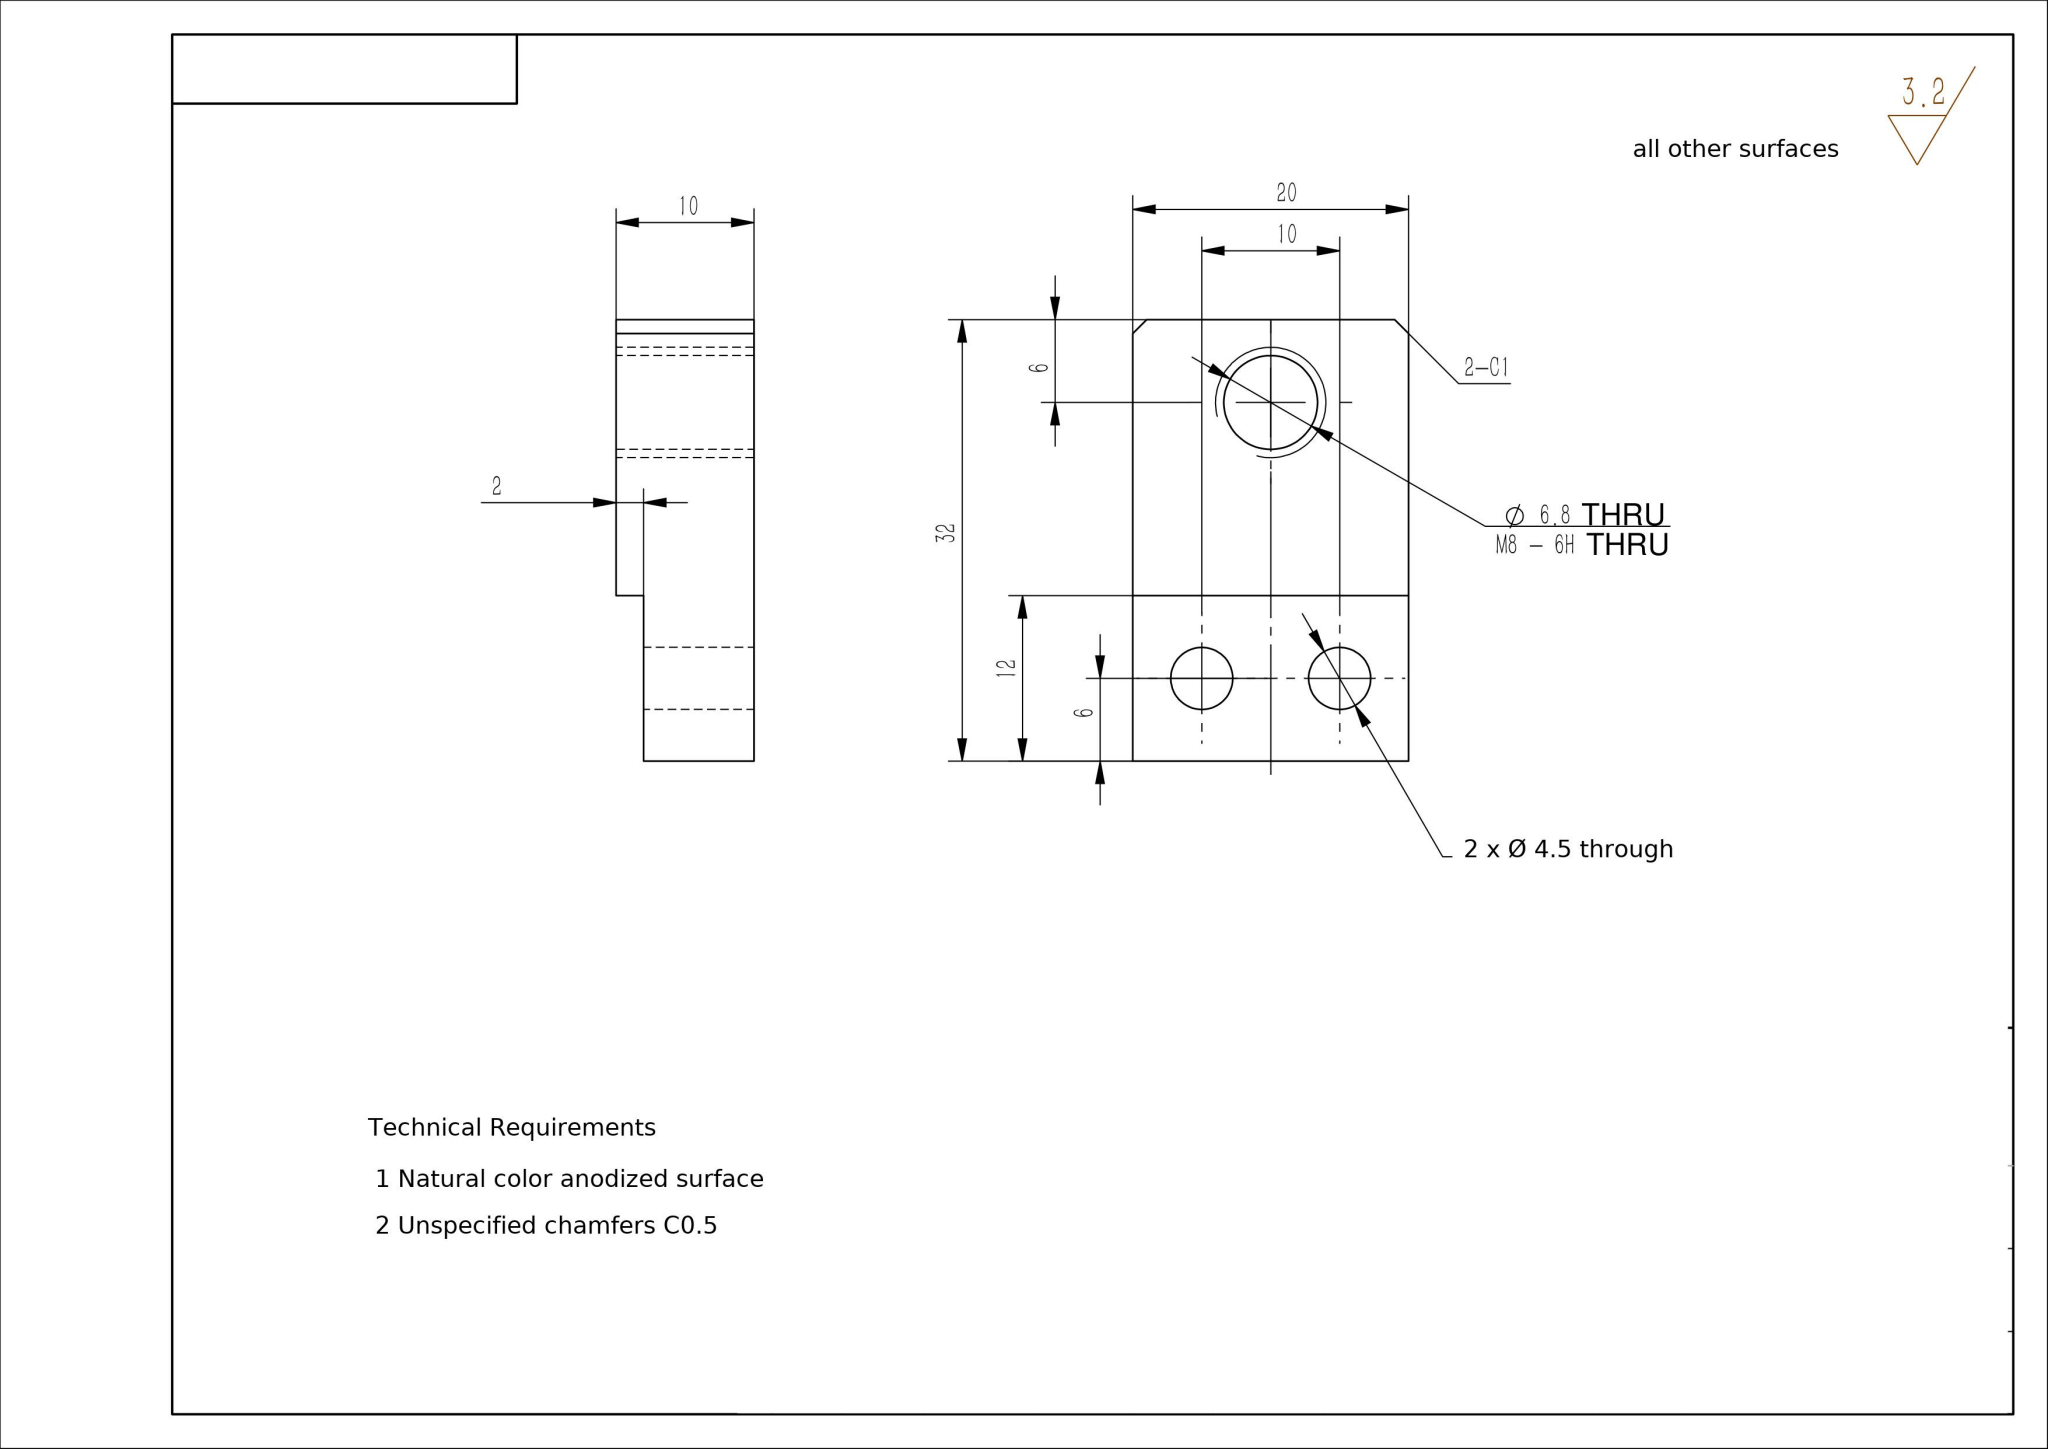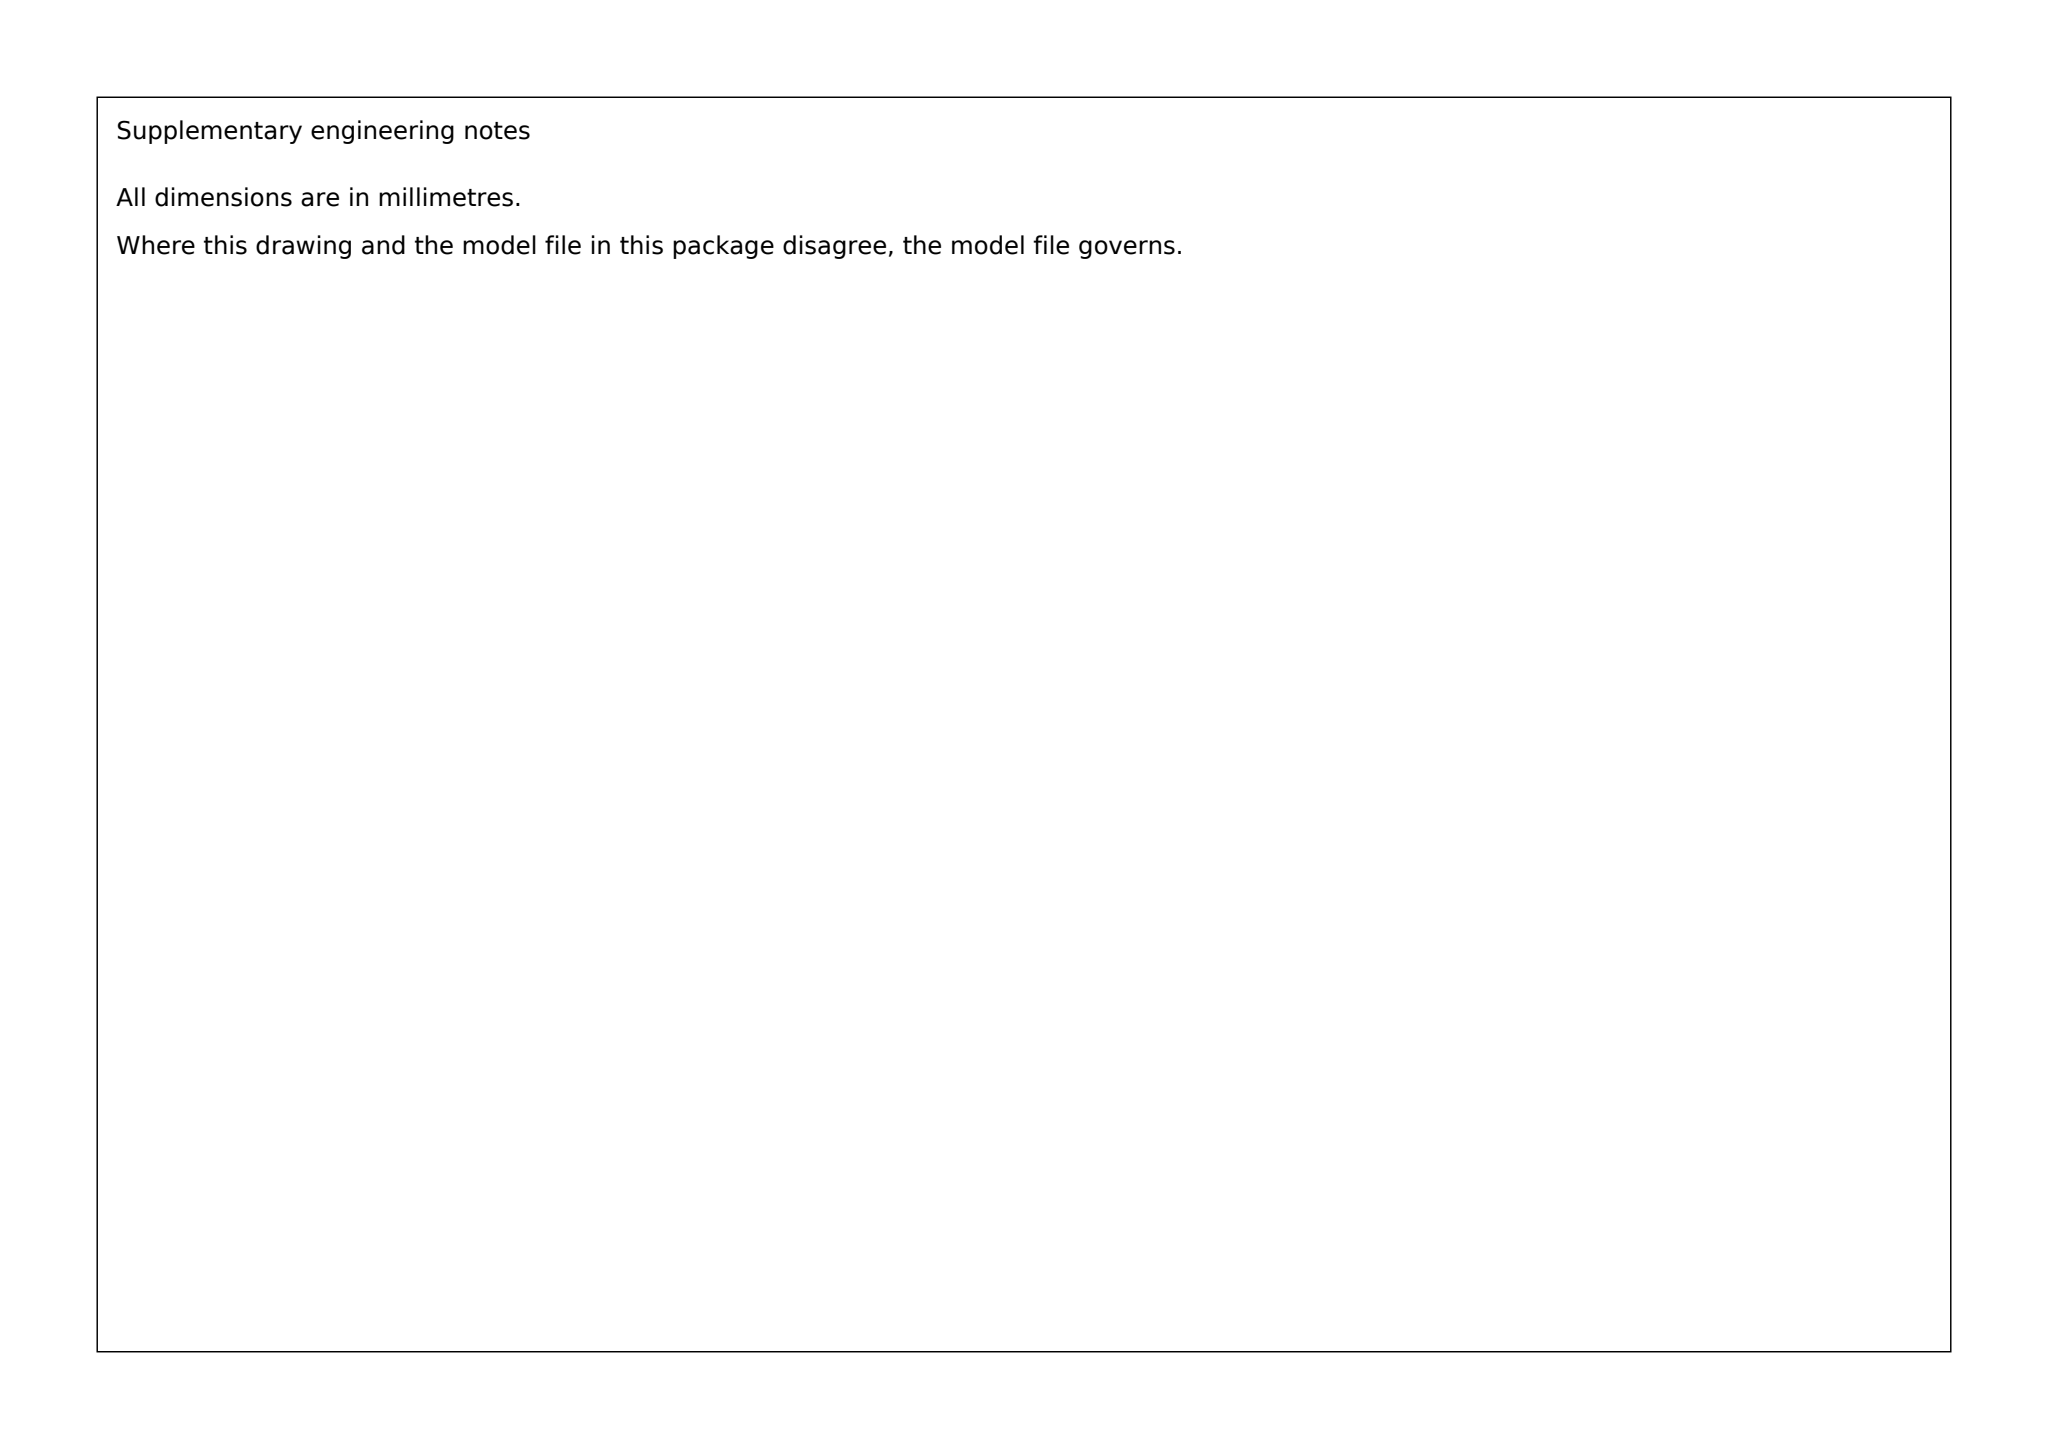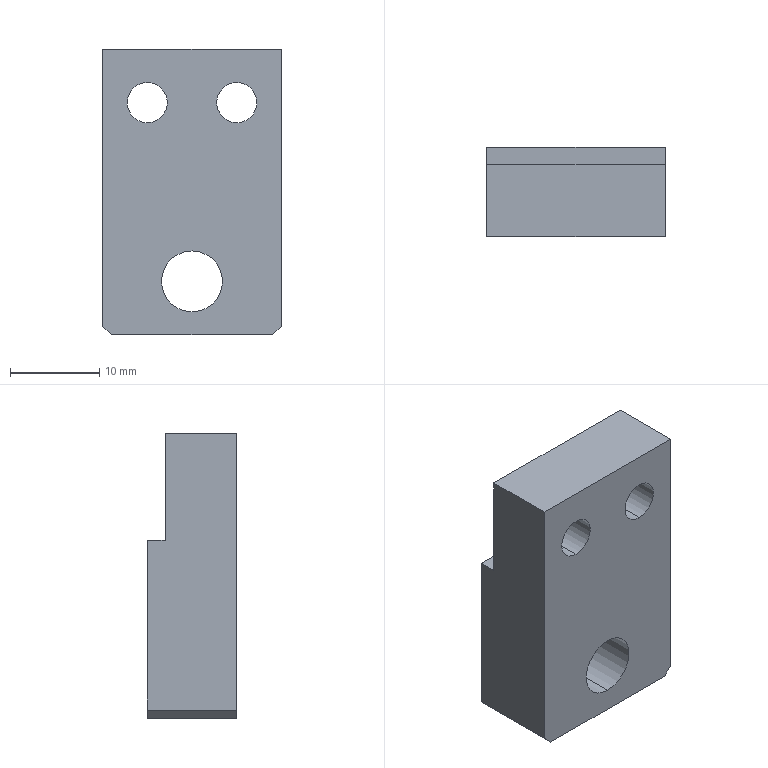Part | SolidWorks | mm | 1 solid | 16 faces | box 20 x 10 x 32 mm | volume 5292 mm3 | plane 10 | cylinder 6 | commonest cylinder face diameters 4.5 x4 6.8 x2
build123d program:
from build123d import *

# Parameters (mm, degrees)
SKETCH1_W                  = 20
SKETCH1_H                  = 32
BOSS_EXTRUDE1_DEPTH        = 10
F_4_5_4_5_DIAMETER_HOLE1_D = 4.5
SKETCH4_W                  = 20
SKETCH4_H                  = 12
CUT_EXTRUDE1_DEPTH         = 2
M8_TAPPED_HOLE1_D          = 6.8
CHAMFER1_SIZE              = 1


with BuildPart() as part:
    # Sketch1 → Boss-Extrude1 (new body)
    with BuildSketch(Plane(origin=(0, 0, 0), x_dir=(1, 0, 0), z_dir=(0, 1, 0))):
        Rectangle(SKETCH1_W, SKETCH1_H)
    extrude(amount=BOSS_EXTRUDE1_DEPTH)

    # 4.5 _4.5_ Diameter Hole1 (through all)
    with Locations(Plane(origin=(0, 10, 0), x_dir=(1, 0, 0), z_dir=(0, 1, 0))):
        with Locations((-5, -10), (5, -10)):
            Hole(F_4_5_4_5_DIAMETER_HOLE1_D / 2)

    # Sketch4 → Cut-Extrude1 (cut)
    with BuildSketch(Plane(origin=(0, 10, 0), x_dir=(1, 0, 0), z_dir=(0, 1, 0))):
        with Locations((0, -10)):
            Rectangle(SKETCH4_W, SKETCH4_H)
    extrude(amount=-CUT_EXTRUDE1_DEPTH, mode=Mode.SUBTRACT)

    # M8 Tapped Hole1 (through all)
    with Locations(Plane(origin=(0, 0, 0), x_dir=(-1, 0, 0), z_dir=(0, -1, 0))):
        with Locations((0, 10)):
            Hole(M8_TAPPED_HOLE1_D / 2)

    # Chamfer1
    chamfer1_edges = [part.edges().sort_by_distance(p)[0] for p in [
        (-10, 5, -16),
        (10, 5, -16),
    ]]
    chamfer(chamfer1_edges, length=CHAMFER1_SIZE)


solid = part.part
STEP:
#1=CARTESIAN_POINT('',(0.,10.,-6.6));
#2=VERTEX_POINT('',#1);
#3=CARTESIAN_POINT('',(0.,10.,-13.4));
#4=VERTEX_POINT('',#3);
#5=CARTESIAN_POINT('',(0.,10.,-10.));
#6=DIRECTION('',(0.,-1.,0.));
#7=DIRECTION('',(0.,0.,-1.));
#8=AXIS2_PLACEMENT_3D('',#5,#6,#7);
#9=CIRCLE('',#8,3.4);
#10=EDGE_CURVE('',#2,#4,#9,.T.);
#11=ORIENTED_EDGE('',*,*,#10,.F.);
#12=CARTESIAN_POINT('',(0.,0.,-6.6));
#13=VERTEX_POINT('',#12);
#14=CARTESIAN_POINT('',(0.,0.,-6.6));
#15=DIRECTION('',(0.,-1.,0.));
#16=VECTOR('',#15,1000.);
#17=LINE('',#14,#16);
#18=EDGE_CURVE('',#2,#13,#17,.T.);
#19=ORIENTED_EDGE('',*,*,#18,.T.);
#20=CARTESIAN_POINT('',(0.,0.,-13.4));
#21=VERTEX_POINT('',#20);
#22=CARTESIAN_POINT('',(0.,0.,-10.));
#23=DIRECTION('',(0.,-1.,0.));
#24=DIRECTION('',(0.,0.,-1.));
#25=AXIS2_PLACEMENT_3D('',#22,#23,#24);
#26=CIRCLE('',#25,3.4);
#27=EDGE_CURVE('',#13,#21,#26,.T.);
#28=ORIENTED_EDGE('',*,*,#27,.T.);
#29=CARTESIAN_POINT('',(0.,0.,-13.4));
#30=DIRECTION('',(0.,-1.,0.));
#31=VECTOR('',#30,1000.);
#32=LINE('',#29,#31);
#33=EDGE_CURVE('',#4,#21,#32,.T.);
#34=ORIENTED_EDGE('',*,*,#33,.F.);
#35=EDGE_LOOP('',(#11,#19,#28,#34));
#36=FACE_OUTER_BOUND('',#35,.T.);
#37=CARTESIAN_POINT('',(0.,0.,-10.));
#38=DIRECTION('',(0.,-1.,0.));
#39=DIRECTION('',(0.,0.,-1.));
#40=AXIS2_PLACEMENT_3D('',#37,#38,#39);
#41=CYLINDRICAL_SURFACE('',#40,3.4);
#42=ADVANCED_FACE('',(#36),#41,.F.);
#43=CARTESIAN_POINT('',(-5.,0.,7.75));
#44=VERTEX_POINT('',#43);
#45=CARTESIAN_POINT('',(-5.,0.,12.25));
#46=VERTEX_POINT('',#45);
#47=CARTESIAN_POINT('',(-5.,0.,10.));
#48=DIRECTION('',(0.,1.,0.));
#49=DIRECTION('',(0.,0.,1.));
#50=AXIS2_PLACEMENT_3D('',#47,#48,#49);
#51=CIRCLE('',#50,2.25);
#52=EDGE_CURVE('',#44,#46,#51,.T.);
#53=ORIENTED_EDGE('',*,*,#52,.F.);
#54=CARTESIAN_POINT('',(-5.,8.,7.75));
#55=VERTEX_POINT('',#54);
#56=CARTESIAN_POINT('',(-5.,10.,7.75));
#57=DIRECTION('',(0.,1.,0.));
#58=VECTOR('',#57,1000.);
#59=LINE('',#56,#58);
#60=EDGE_CURVE('',#44,#55,#59,.T.);
#61=ORIENTED_EDGE('',*,*,#60,.T.);
#62=CARTESIAN_POINT('',(-5.,8.,12.25));
#63=VERTEX_POINT('',#62);
#64=CARTESIAN_POINT('',(-5.,8.,10.));
#65=DIRECTION('',(0.,-1.,0.));
#66=DIRECTION('',(0.,0.,1.));
#67=AXIS2_PLACEMENT_3D('',#64,#65,#66);
#68=CIRCLE('',#67,2.25);
#69=EDGE_CURVE('',#63,#55,#68,.T.);
#70=ORIENTED_EDGE('',*,*,#69,.F.);
#71=CARTESIAN_POINT('',(-5.,10.,12.25));
#72=DIRECTION('',(0.,1.,0.));
#73=VECTOR('',#72,1000.);
#74=LINE('',#71,#73);
#75=EDGE_CURVE('',#46,#63,#74,.T.);
#76=ORIENTED_EDGE('',*,*,#75,.F.);
#77=EDGE_LOOP('',(#53,#61,#70,#76));
#78=FACE_OUTER_BOUND('',#77,.T.);
#79=CARTESIAN_POINT('',(-5.,10.,10.));
#80=DIRECTION('',(0.,1.,0.));
#81=DIRECTION('',(0.,0.,1.));
#82=AXIS2_PLACEMENT_3D('',#79,#80,#81);
#83=CYLINDRICAL_SURFACE('',#82,2.25);
#84=ADVANCED_FACE('',(#78),#83,.F.);
#85=CARTESIAN_POINT('',(5.,0.,7.75));
#86=VERTEX_POINT('',#85);
#87=CARTESIAN_POINT('',(5.,0.,12.25));
#88=VERTEX_POINT('',#87);
#89=CARTESIAN_POINT('',(5.,0.,10.));
#90=DIRECTION('',(0.,1.,0.));
#91=DIRECTION('',(0.,0.,1.));
#92=AXIS2_PLACEMENT_3D('',#89,#90,#91);
#93=CIRCLE('',#92,2.25);
#94=EDGE_CURVE('',#86,#88,#93,.T.);
#95=ORIENTED_EDGE('',*,*,#94,.F.);
#96=CARTESIAN_POINT('',(5.,8.,7.75));
#97=VERTEX_POINT('',#96);
#98=CARTESIAN_POINT('',(5.,10.,7.75));
#99=DIRECTION('',(0.,1.,0.));
#100=VECTOR('',#99,1000.);
#101=LINE('',#98,#100);
#102=EDGE_CURVE('',#86,#97,#101,.T.);
#103=ORIENTED_EDGE('',*,*,#102,.T.);
#104=CARTESIAN_POINT('',(5.,8.,12.25));
#105=VERTEX_POINT('',#104);
#106=CARTESIAN_POINT('',(5.,8.,10.));
#107=DIRECTION('',(0.,-1.,0.));
#108=DIRECTION('',(0.,0.,1.));
#109=AXIS2_PLACEMENT_3D('',#106,#107,#108);
#110=CIRCLE('',#109,2.25);
#111=EDGE_CURVE('',#105,#97,#110,.T.);
#112=ORIENTED_EDGE('',*,*,#111,.F.);
#113=CARTESIAN_POINT('',(5.,10.,12.25));
#114=DIRECTION('',(0.,1.,0.));
#115=VECTOR('',#114,1000.);
#116=LINE('',#113,#115);
#117=EDGE_CURVE('',#88,#105,#116,.T.);
#118=ORIENTED_EDGE('',*,*,#117,.F.);
#119=EDGE_LOOP('',(#95,#103,#112,#118));
#120=FACE_OUTER_BOUND('',#119,.T.);
#121=CARTESIAN_POINT('',(5.,10.,10.));
#122=DIRECTION('',(0.,1.,0.));
#123=DIRECTION('',(0.,0.,1.));
#124=AXIS2_PLACEMENT_3D('',#121,#122,#123);
#125=CYLINDRICAL_SURFACE('',#124,2.25);
#126=ADVANCED_FACE('',(#120),#125,.F.);
#127=CARTESIAN_POINT('',(-10.,8.,16.));
#128=VERTEX_POINT('',#127);
#129=CARTESIAN_POINT('',(10.,8.,16.));
#130=VERTEX_POINT('',#129);
#131=CARTESIAN_POINT('',(-10.,8.,16.));
#132=DIRECTION('',(1.,0.,0.));
#133=VECTOR('',#132,1000.);
#134=LINE('',#131,#133);
#135=EDGE_CURVE('',#128,#130,#134,.T.);
#136=ORIENTED_EDGE('',*,*,#135,.F.);
#137=CARTESIAN_POINT('',(-10.,0.,16.));
#138=VERTEX_POINT('',#137);
#139=CARTESIAN_POINT('',(-10.,10.,16.));
#140=DIRECTION('',(0.,-1.,0.));
#141=VECTOR('',#140,1000.);
#142=LINE('',#139,#141);
#143=EDGE_CURVE('',#128,#138,#142,.T.);
#144=ORIENTED_EDGE('',*,*,#143,.T.);
#145=CARTESIAN_POINT('',(10.,0.,16.));
#146=VERTEX_POINT('',#145);
#147=CARTESIAN_POINT('',(-10.,0.,16.));
#148=DIRECTION('',(1.,0.,0.));
#149=VECTOR('',#148,1000.);
#150=LINE('',#147,#149);
#151=EDGE_CURVE('',#138,#146,#150,.T.);
#152=ORIENTED_EDGE('',*,*,#151,.T.);
#153=CARTESIAN_POINT('',(10.,10.,16.));
#154=DIRECTION('',(0.,-1.,0.));
#155=VECTOR('',#154,1000.);
#156=LINE('',#153,#155);
#157=EDGE_CURVE('',#130,#146,#156,.T.);
#158=ORIENTED_EDGE('',*,*,#157,.F.);
#159=EDGE_LOOP('',(#136,#144,#152,#158));
#160=FACE_OUTER_BOUND('',#159,.T.);
#161=CARTESIAN_POINT('',(-10.,10.,16.));
#162=DIRECTION('',(0.,0.,-1.));
#163=DIRECTION('',(-1.,0.,0.));
#164=AXIS2_PLACEMENT_3D('',#161,#162,#163);
#165=PLANE('',#164);
#166=ADVANCED_FACE('',(#160),#165,.F.);
#167=ORIENTED_EDGE('',*,*,#102,.F.);
#168=CARTESIAN_POINT('',(5.,0.,10.));
#169=DIRECTION('',(0.,1.,0.));
#170=DIRECTION('',(0.,0.,1.));
#171=AXIS2_PLACEMENT_3D('',#168,#169,#170);
#172=CIRCLE('',#171,2.25);
#173=EDGE_CURVE('',#88,#86,#172,.T.);
#174=ORIENTED_EDGE('',*,*,#173,.F.);
#175=ORIENTED_EDGE('',*,*,#117,.T.);
#176=CARTESIAN_POINT('',(5.,8.,10.));
#177=DIRECTION('',(0.,-1.,0.));
#178=DIRECTION('',(0.,0.,1.));
#179=AXIS2_PLACEMENT_3D('',#176,#177,#178);
#180=CIRCLE('',#179,2.25);
#181=EDGE_CURVE('',#97,#105,#180,.T.);
#182=ORIENTED_EDGE('',*,*,#181,.F.);
#183=EDGE_LOOP('',(#167,#174,#175,#182));
#184=FACE_OUTER_BOUND('',#183,.T.);
#185=CARTESIAN_POINT('',(5.,10.,10.));
#186=DIRECTION('',(0.,1.,0.));
#187=DIRECTION('',(0.,0.,1.));
#188=AXIS2_PLACEMENT_3D('',#185,#186,#187);
#189=CYLINDRICAL_SURFACE('',#188,2.25);
#190=ADVANCED_FACE('',(#184),#189,.F.);
#191=ORIENTED_EDGE('',*,*,#60,.F.);
#192=CARTESIAN_POINT('',(-5.,0.,10.));
#193=DIRECTION('',(0.,1.,0.));
#194=DIRECTION('',(0.,0.,1.));
#195=AXIS2_PLACEMENT_3D('',#192,#193,#194);
#196=CIRCLE('',#195,2.25);
#197=EDGE_CURVE('',#46,#44,#196,.T.);
#198=ORIENTED_EDGE('',*,*,#197,.F.);
#199=ORIENTED_EDGE('',*,*,#75,.T.);
#200=CARTESIAN_POINT('',(-5.,8.,10.));
#201=DIRECTION('',(0.,-1.,0.));
#202=DIRECTION('',(0.,0.,1.));
#203=AXIS2_PLACEMENT_3D('',#200,#201,#202);
#204=CIRCLE('',#203,2.25);
#205=EDGE_CURVE('',#55,#63,#204,.T.);
#206=ORIENTED_EDGE('',*,*,#205,.F.);
#207=EDGE_LOOP('',(#191,#198,#199,#206));
#208=FACE_OUTER_BOUND('',#207,.T.);
#209=CARTESIAN_POINT('',(-5.,10.,10.));
#210=DIRECTION('',(0.,1.,0.));
#211=DIRECTION('',(0.,0.,1.));
#212=AXIS2_PLACEMENT_3D('',#209,#210,#211);
#213=CYLINDRICAL_SURFACE('',#212,2.25);
#214=ADVANCED_FACE('',(#208),#213,.F.);
#215=CARTESIAN_POINT('',(10.,0.,-15.));
#216=VERTEX_POINT('',#215);
#217=CARTESIAN_POINT('',(10.,0.,16.));
#218=DIRECTION('',(0.,0.,-1.));
#219=VECTOR('',#218,1000.);
#220=LINE('',#217,#219);
#221=EDGE_CURVE('',#146,#216,#220,.T.);
#222=ORIENTED_EDGE('',*,*,#221,.T.);
#223=CARTESIAN_POINT('',(10.,10.,-15.));
#224=VERTEX_POINT('',#223);
#225=CARTESIAN_POINT('',(10.,10.,-15.));
#226=DIRECTION('',(0.,1.,0.));
#227=VECTOR('',#226,1000.);
#228=LINE('',#225,#227);
#229=EDGE_CURVE('',#216,#224,#228,.T.);
#230=ORIENTED_EDGE('',*,*,#229,.T.);
#231=CARTESIAN_POINT('',(10.,10.,4.));
#232=VERTEX_POINT('',#231);
#233=CARTESIAN_POINT('',(10.,10.,16.));
#234=DIRECTION('',(0.,0.,-1.));
#235=VECTOR('',#234,1000.);
#236=LINE('',#233,#235);
#237=EDGE_CURVE('',#232,#224,#236,.T.);
#238=ORIENTED_EDGE('',*,*,#237,.F.);
#239=CARTESIAN_POINT('',(10.,8.,4.));
#240=VERTEX_POINT('',#239);
#241=CARTESIAN_POINT('',(10.,8.,4.));
#242=DIRECTION('',(0.,1.,0.));
#243=VECTOR('',#242,1000.);
#244=LINE('',#241,#243);
#245=EDGE_CURVE('',#240,#232,#244,.T.);
#246=ORIENTED_EDGE('',*,*,#245,.F.);
#247=CARTESIAN_POINT('',(10.,8.,4.));
#248=DIRECTION('',(0.,0.,-1.));
#249=VECTOR('',#248,1000.);
#250=LINE('',#247,#249);
#251=EDGE_CURVE('',#130,#240,#250,.T.);
#252=ORIENTED_EDGE('',*,*,#251,.F.);
#253=ORIENTED_EDGE('',*,*,#157,.T.);
#254=EDGE_LOOP('',(#222,#230,#238,#246,#252,#253));
#255=FACE_OUTER_BOUND('',#254,.T.);
#256=CARTESIAN_POINT('',(10.,10.,16.));
#257=DIRECTION('',(-1.,0.,0.));
#258=DIRECTION('',(0.,0.,1.));
#259=AXIS2_PLACEMENT_3D('',#256,#257,#258);
#260=PLANE('',#259);
#261=ADVANCED_FACE('',(#255),#260,.F.);
#262=CARTESIAN_POINT('',(9.,0.,-16.));
#263=VERTEX_POINT('',#262);
#264=CARTESIAN_POINT('',(-9.,0.,-16.));
#265=VERTEX_POINT('',#264);
#266=CARTESIAN_POINT('',(-10.,0.,-16.));
#267=DIRECTION('',(-1.,0.,0.));
#268=VECTOR('',#267,1000.);
#269=LINE('',#266,#268);
#270=EDGE_CURVE('',#263,#265,#269,.T.);
#271=ORIENTED_EDGE('',*,*,#270,.T.);
#272=CARTESIAN_POINT('',(-9.,10.,-16.));
#273=VERTEX_POINT('',#272);
#274=CARTESIAN_POINT('',(-9.,10.,-16.));
#275=DIRECTION('',(0.,1.,0.));
#276=VECTOR('',#275,1000.);
#277=LINE('',#274,#276);
#278=EDGE_CURVE('',#265,#273,#277,.T.);
#279=ORIENTED_EDGE('',*,*,#278,.T.);
#280=CARTESIAN_POINT('',(9.,10.,-16.));
#281=VERTEX_POINT('',#280);
#282=CARTESIAN_POINT('',(-10.,10.,-16.));
#283=DIRECTION('',(-1.,0.,0.));
#284=VECTOR('',#283,1000.);
#285=LINE('',#282,#284);
#286=EDGE_CURVE('',#281,#273,#285,.T.);
#287=ORIENTED_EDGE('',*,*,#286,.F.);
#288=CARTESIAN_POINT('',(9.,10.,-16.));
#289=DIRECTION('',(0.,-1.,0.));
#290=VECTOR('',#289,1000.);
#291=LINE('',#288,#290);
#292=EDGE_CURVE('',#281,#263,#291,.T.);
#293=ORIENTED_EDGE('',*,*,#292,.T.);
#294=EDGE_LOOP('',(#271,#279,#287,#293));
#295=FACE_OUTER_BOUND('',#294,.T.);
#296=CARTESIAN_POINT('',(-10.,10.,-16.));
#297=DIRECTION('',(0.,0.,1.));
#298=DIRECTION('',(1.,0.,0.));
#299=AXIS2_PLACEMENT_3D('',#296,#297,#298);
#300=PLANE('',#299);
#301=ADVANCED_FACE('',(#295),#300,.F.);
#302=CARTESIAN_POINT('',(-10.,10.,-15.));
#303=VERTEX_POINT('',#302);
#304=CARTESIAN_POINT('',(-10.,10.,4.));
#305=VERTEX_POINT('',#304);
#306=CARTESIAN_POINT('',(-10.,10.,16.));
#307=DIRECTION('',(0.,0.,1.));
#308=VECTOR('',#307,1000.);
#309=LINE('',#306,#308);
#310=EDGE_CURVE('',#303,#305,#309,.T.);
#311=ORIENTED_EDGE('',*,*,#310,.F.);
#312=CARTESIAN_POINT('',(-10.,0.,-15.));
#313=VERTEX_POINT('',#312);
#314=CARTESIAN_POINT('',(-10.,10.,-15.));
#315=DIRECTION('',(0.,-1.,0.));
#316=VECTOR('',#315,1000.);
#317=LINE('',#314,#316);
#318=EDGE_CURVE('',#303,#313,#317,.T.);
#319=ORIENTED_EDGE('',*,*,#318,.T.);
#320=CARTESIAN_POINT('',(-10.,0.,16.));
#321=DIRECTION('',(0.,0.,1.));
#322=VECTOR('',#321,1000.);
#323=LINE('',#320,#322);
#324=EDGE_CURVE('',#313,#138,#323,.T.);
#325=ORIENTED_EDGE('',*,*,#324,.T.);
#326=ORIENTED_EDGE('',*,*,#143,.F.);
#327=CARTESIAN_POINT('',(-10.,8.,4.));
#328=VERTEX_POINT('',#327);
#329=CARTESIAN_POINT('',(-10.,8.,4.));
#330=DIRECTION('',(0.,0.,1.));
#331=VECTOR('',#330,1000.);
#332=LINE('',#329,#331);
#333=EDGE_CURVE('',#328,#128,#332,.T.);
#334=ORIENTED_EDGE('',*,*,#333,.F.);
#335=CARTESIAN_POINT('',(-10.,8.,4.));
#336=DIRECTION('',(0.,1.,0.));
#337=VECTOR('',#336,1000.);
#338=LINE('',#335,#337);
#339=EDGE_CURVE('',#328,#305,#338,.T.);
#340=ORIENTED_EDGE('',*,*,#339,.T.);
#341=EDGE_LOOP('',(#311,#319,#325,#326,#334,#340));
#342=FACE_OUTER_BOUND('',#341,.T.);
#343=CARTESIAN_POINT('',(-10.,10.,16.));
#344=DIRECTION('',(1.,0.,0.));
#345=DIRECTION('',(0.,0.,-1.));
#346=AXIS2_PLACEMENT_3D('',#343,#344,#345);
#347=PLANE('',#346);
#348=ADVANCED_FACE('',(#342),#347,.F.);
#349=CARTESIAN_POINT('',(0.,10.,-10.));
#350=DIRECTION('',(0.,-1.,0.));
#351=DIRECTION('',(0.,0.,-1.));
#352=AXIS2_PLACEMENT_3D('',#349,#350,#351);
#353=CIRCLE('',#352,3.4);
#354=EDGE_CURVE('',#4,#2,#353,.T.);
#355=ORIENTED_EDGE('',*,*,#354,.T.);
#356=ORIENTED_EDGE('',*,*,#10,.T.);
#357=EDGE_LOOP('',(#355,#356));
#358=FACE_BOUND('',#357,.T.);
#359=ORIENTED_EDGE('',*,*,#286,.T.);
#360=CARTESIAN_POINT('',(-10.,10.,-15.));
#361=DIRECTION('',(-0.7071,0.,0.7071));
#362=VECTOR('',#361,1000.);
#363=LINE('',#360,#362);
#364=EDGE_CURVE('',#273,#303,#363,.T.);
#365=ORIENTED_EDGE('',*,*,#364,.T.);
#366=ORIENTED_EDGE('',*,*,#310,.T.);
#367=CARTESIAN_POINT('',(-10.,10.,4.));
#368=DIRECTION('',(-1.,0.,0.));
#369=VECTOR('',#368,1000.);
#370=LINE('',#367,#369);
#371=EDGE_CURVE('',#232,#305,#370,.T.);
#372=ORIENTED_EDGE('',*,*,#371,.F.);
#373=ORIENTED_EDGE('',*,*,#237,.T.);
#374=CARTESIAN_POINT('',(9.,10.,-16.));
#375=DIRECTION('',(-0.7071,0.,-0.7071));
#376=VECTOR('',#375,1000.);
#377=LINE('',#374,#376);
#378=EDGE_CURVE('',#224,#281,#377,.T.);
#379=ORIENTED_EDGE('',*,*,#378,.T.);
#380=EDGE_LOOP('',(#359,#365,#366,#372,#373,#379));
#381=FACE_OUTER_BOUND('',#380,.T.);
#382=CARTESIAN_POINT('',(0.,10.,0.));
#383=DIRECTION('',(0.,-1.,0.));
#384=DIRECTION('',(0.,0.,-1.));
#385=AXIS2_PLACEMENT_3D('',#382,#383,#384);
#386=PLANE('',#385);
#387=ADVANCED_FACE('',(#358,#381),#386,.F.);
#388=CARTESIAN_POINT('',(0.,0.,-10.));
#389=DIRECTION('',(0.,-1.,0.));
#390=DIRECTION('',(0.,0.,-1.));
#391=AXIS2_PLACEMENT_3D('',#388,#389,#390);
#392=CIRCLE('',#391,3.4);
#393=EDGE_CURVE('',#21,#13,#392,.T.);
#394=ORIENTED_EDGE('',*,*,#393,.F.);
#395=ORIENTED_EDGE('',*,*,#27,.F.);
#396=EDGE_LOOP('',(#394,#395));
#397=FACE_BOUND('',#396,.T.);
#398=ORIENTED_EDGE('',*,*,#197,.T.);
#399=ORIENTED_EDGE('',*,*,#52,.T.);
#400=EDGE_LOOP('',(#398,#399));
#401=FACE_BOUND('',#400,.T.);
#402=ORIENTED_EDGE('',*,*,#173,.T.);
#403=ORIENTED_EDGE('',*,*,#94,.T.);
#404=EDGE_LOOP('',(#402,#403));
#405=FACE_BOUND('',#404,.T.);
#406=ORIENTED_EDGE('',*,*,#324,.F.);
#407=CARTESIAN_POINT('',(-12.5,0.,-12.5));
#408=DIRECTION('',(0.7071,0.,-0.7071));
#409=VECTOR('',#408,1000.);
#410=LINE('',#407,#409);
#411=EDGE_CURVE('',#313,#265,#410,.T.);
#412=ORIENTED_EDGE('',*,*,#411,.T.);
#413=ORIENTED_EDGE('',*,*,#270,.F.);
#414=CARTESIAN_POINT('',(12.5,0.,-12.5));
#415=DIRECTION('',(0.7071,0.,0.7071));
#416=VECTOR('',#415,1000.);
#417=LINE('',#414,#416);
#418=EDGE_CURVE('',#263,#216,#417,.T.);
#419=ORIENTED_EDGE('',*,*,#418,.T.);
#420=ORIENTED_EDGE('',*,*,#221,.F.);
#421=ORIENTED_EDGE('',*,*,#151,.F.);
#422=EDGE_LOOP('',(#406,#412,#413,#419,#420,#421));
#423=FACE_OUTER_BOUND('',#422,.T.);
#424=CARTESIAN_POINT('',(0.,0.,0.));
#425=DIRECTION('',(0.,-1.,0.));
#426=DIRECTION('',(0.,0.,-1.));
#427=AXIS2_PLACEMENT_3D('',#424,#425,#426);
#428=PLANE('',#427);
#429=ADVANCED_FACE('',(#397,#401,#405,#423),#428,.T.);
#430=ORIENTED_EDGE('',*,*,#333,.T.);
#431=ORIENTED_EDGE('',*,*,#135,.T.);
#432=ORIENTED_EDGE('',*,*,#251,.T.);
#433=CARTESIAN_POINT('',(-10.,8.,4.));
#434=DIRECTION('',(-1.,0.,0.));
#435=VECTOR('',#434,1000.);
#436=LINE('',#433,#435);
#437=EDGE_CURVE('',#240,#328,#436,.T.);
#438=ORIENTED_EDGE('',*,*,#437,.T.);
#439=EDGE_LOOP('',(#430,#431,#432,#438));
#440=FACE_OUTER_BOUND('',#439,.T.);
#441=ORIENTED_EDGE('',*,*,#69,.T.);
#442=ORIENTED_EDGE('',*,*,#205,.T.);
#443=EDGE_LOOP('',(#441,#442));
#444=FACE_BOUND('',#443,.T.);
#445=ORIENTED_EDGE('',*,*,#111,.T.);
#446=ORIENTED_EDGE('',*,*,#181,.T.);
#447=EDGE_LOOP('',(#445,#446));
#448=FACE_BOUND('',#447,.T.);
#449=CARTESIAN_POINT('',(0.,8.,0.));
#450=DIRECTION('',(0.,1.,0.));
#451=DIRECTION('',(0.,0.,1.));
#452=AXIS2_PLACEMENT_3D('',#449,#450,#451);
#453=PLANE('',#452);
#454=ADVANCED_FACE('',(#440,#444,#448),#453,.T.);
#455=ORIENTED_EDGE('',*,*,#371,.T.);
#456=ORIENTED_EDGE('',*,*,#339,.F.);
#457=ORIENTED_EDGE('',*,*,#437,.F.);
#458=ORIENTED_EDGE('',*,*,#245,.T.);
#459=EDGE_LOOP('',(#455,#456,#457,#458));
#460=FACE_OUTER_BOUND('',#459,.T.);
#461=CARTESIAN_POINT('',(-10.,8.,4.));
#462=DIRECTION('',(0.,0.,-1.));
#463=DIRECTION('',(-1.,0.,0.));
#464=AXIS2_PLACEMENT_3D('',#461,#462,#463);
#465=PLANE('',#464);
#466=ADVANCED_FACE('',(#460),#465,.F.);
#467=ORIENTED_EDGE('',*,*,#18,.F.);
#468=ORIENTED_EDGE('',*,*,#354,.F.);
#469=ORIENTED_EDGE('',*,*,#33,.T.);
#470=ORIENTED_EDGE('',*,*,#393,.T.);
#471=EDGE_LOOP('',(#467,#468,#469,#470));
#472=FACE_OUTER_BOUND('',#471,.T.);
#473=CARTESIAN_POINT('',(0.,0.,-10.));
#474=DIRECTION('',(0.,-1.,0.));
#475=DIRECTION('',(0.,0.,-1.));
#476=AXIS2_PLACEMENT_3D('',#473,#474,#475);
#477=CYLINDRICAL_SURFACE('',#476,3.4);
#478=ADVANCED_FACE('',(#472),#477,.F.);
#479=ORIENTED_EDGE('',*,*,#364,.F.);
#480=ORIENTED_EDGE('',*,*,#278,.F.);
#481=ORIENTED_EDGE('',*,*,#411,.F.);
#482=ORIENTED_EDGE('',*,*,#318,.F.);
#483=EDGE_LOOP('',(#479,#480,#481,#482));
#484=FACE_OUTER_BOUND('',#483,.T.);
#485=CARTESIAN_POINT('',(-10.,10.,-15.));
#486=DIRECTION('',(0.7071,0.,0.7071));
#487=DIRECTION('',(0.,-1.,0.));
#488=AXIS2_PLACEMENT_3D('',#485,#486,#487);
#489=PLANE('',#488);
#490=ADVANCED_FACE('',(#484),#489,.F.);
#491=ORIENTED_EDGE('',*,*,#378,.F.);
#492=ORIENTED_EDGE('',*,*,#229,.F.);
#493=ORIENTED_EDGE('',*,*,#418,.F.);
#494=ORIENTED_EDGE('',*,*,#292,.F.);
#495=EDGE_LOOP('',(#491,#492,#493,#494));
#496=FACE_OUTER_BOUND('',#495,.T.);
#497=CARTESIAN_POINT('',(9.,10.,-16.));
#498=DIRECTION('',(-0.7071,0.,0.7071));
#499=DIRECTION('',(0.,-1.,0.));
#500=AXIS2_PLACEMENT_3D('',#497,#498,#499);
#501=PLANE('',#500);
#502=ADVANCED_FACE('',(#496),#501,.F.);
#503=CLOSED_SHELL('',(#42,#84,#126,#166,#190,#214,#261,#301,#348,#387,#429,#454,#466,#478,#490,#502));
#504=MANIFOLD_SOLID_BREP('',#503);
#505=CARTESIAN_POINT('',(0.,0.,0.));
#506=DIRECTION('',(0.,0.,1.));
#507=DIRECTION('',(1.,0.,0.));
#508=AXIS2_PLACEMENT_3D('',#505,#506,#507);
#509=(LENGTH_UNIT()NAMED_UNIT(*)SI_UNIT(.MILLI.,.METRE.));
#510=UNCERTAINTY_MEASURE_WITH_UNIT(LENGTH_MEASURE(0.00001),#509,'','');
#511=(NAMED_UNIT(*)PLANE_ANGLE_UNIT()SI_UNIT($,.RADIAN.));
#512=(NAMED_UNIT(*)SI_UNIT($,.STERADIAN.)SOLID_ANGLE_UNIT());
#513=(GEOMETRIC_REPRESENTATION_CONTEXT(3)GLOBAL_UNCERTAINTY_ASSIGNED_CONTEXT((#510))GLOBAL_UNIT_ASSIGNED_CONTEXT((#509,#511,#512))REPRESENTATION_CONTEXT('',''));
#514=ADVANCED_BREP_SHAPE_REPRESENTATION('',(#504,#508),#513);